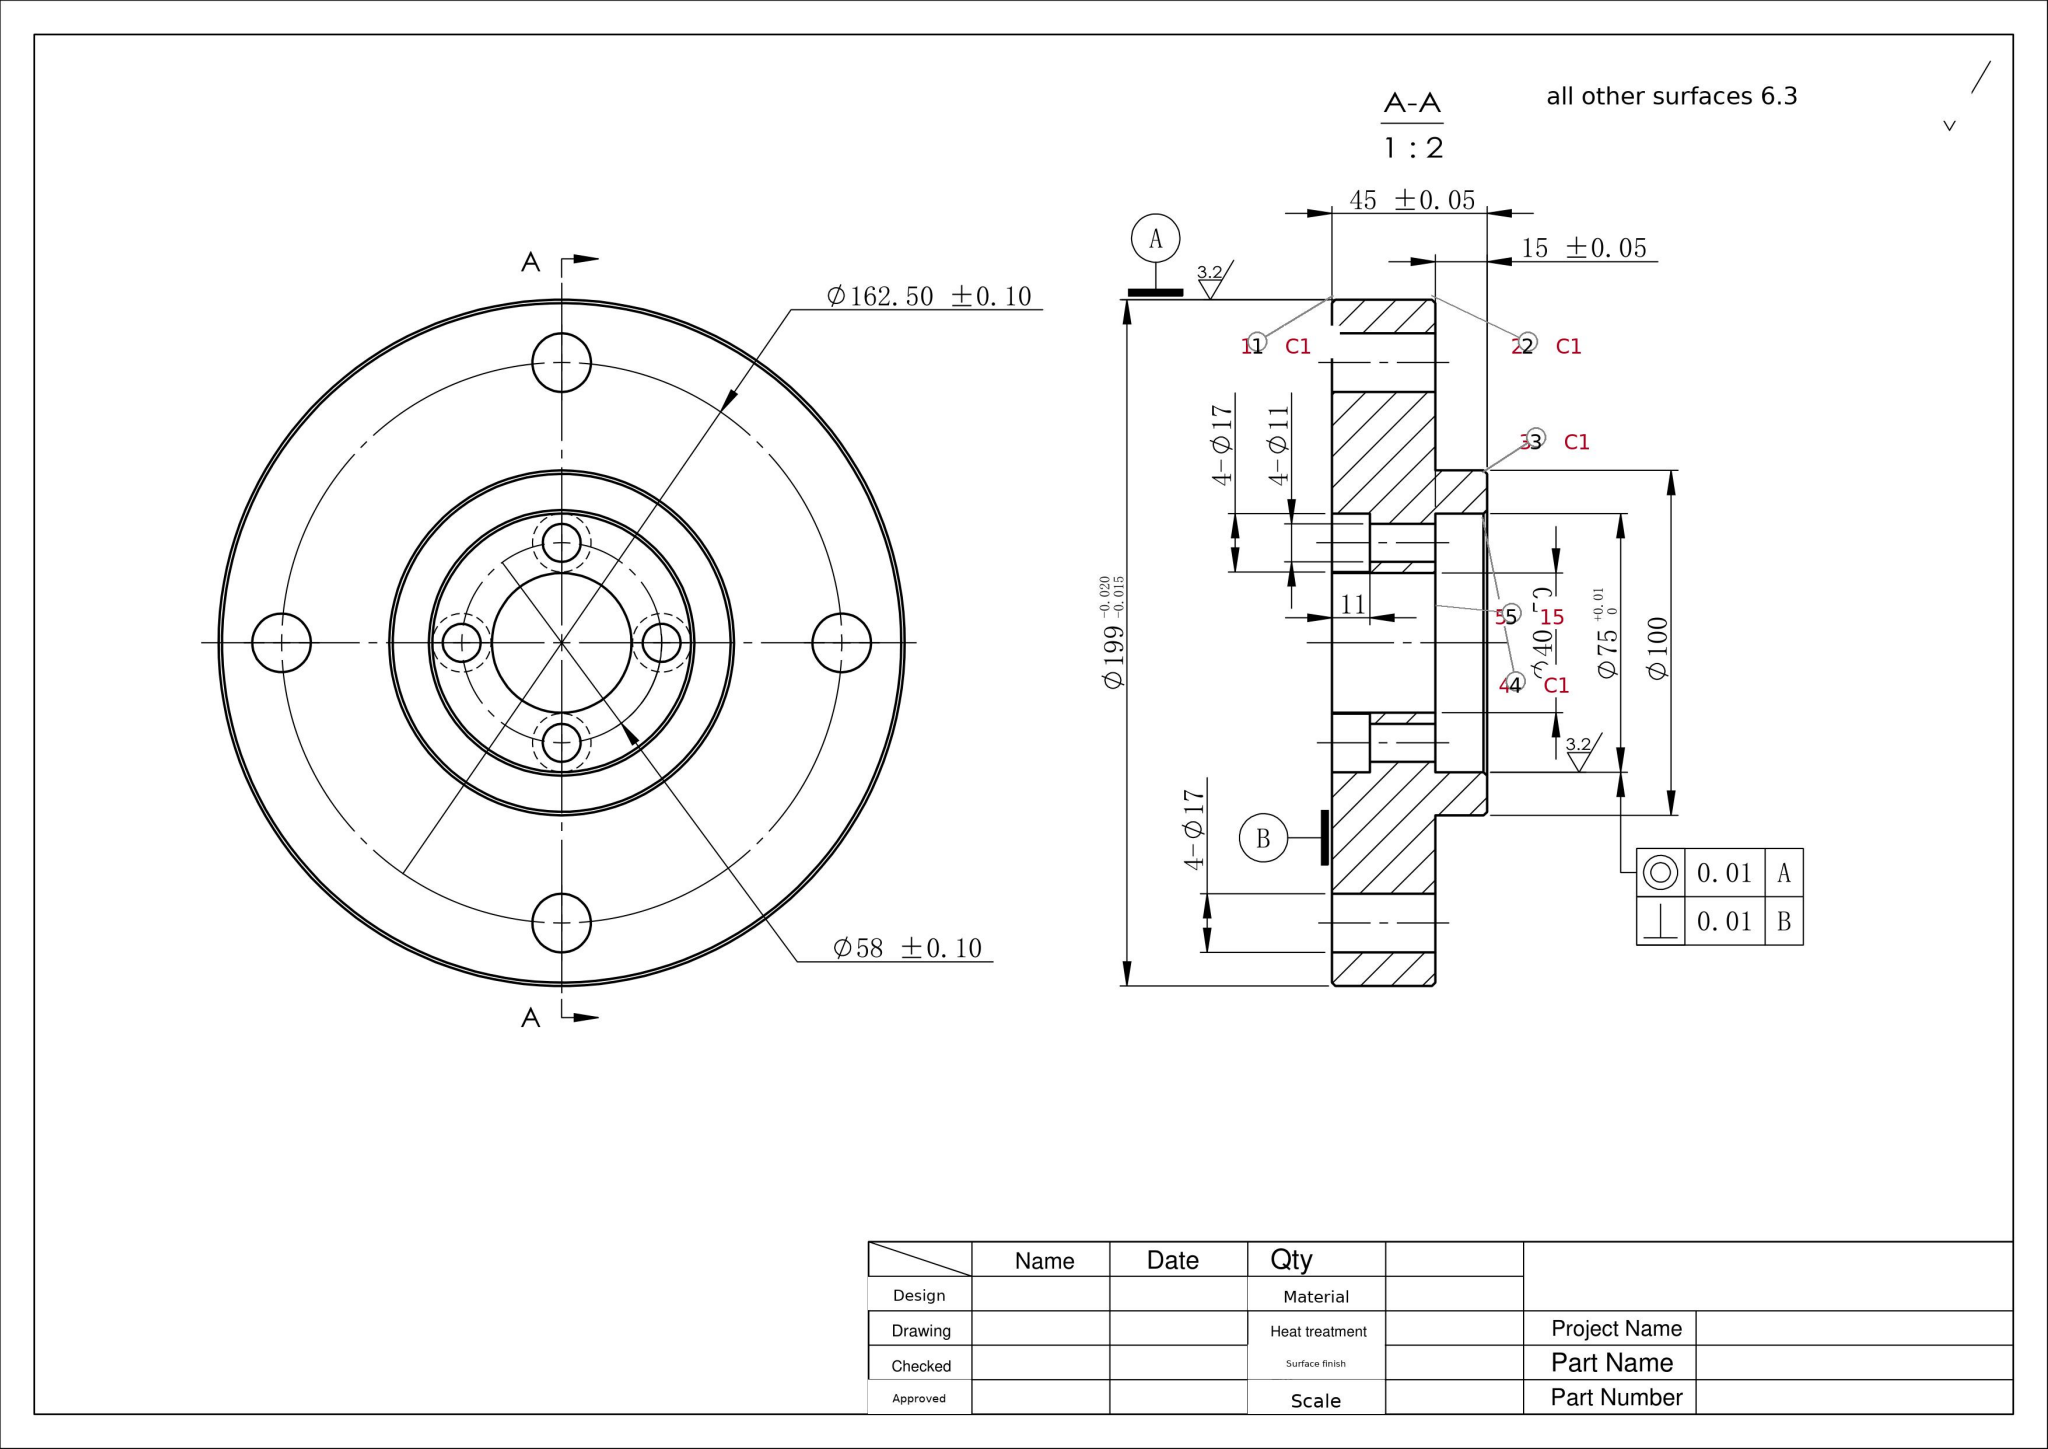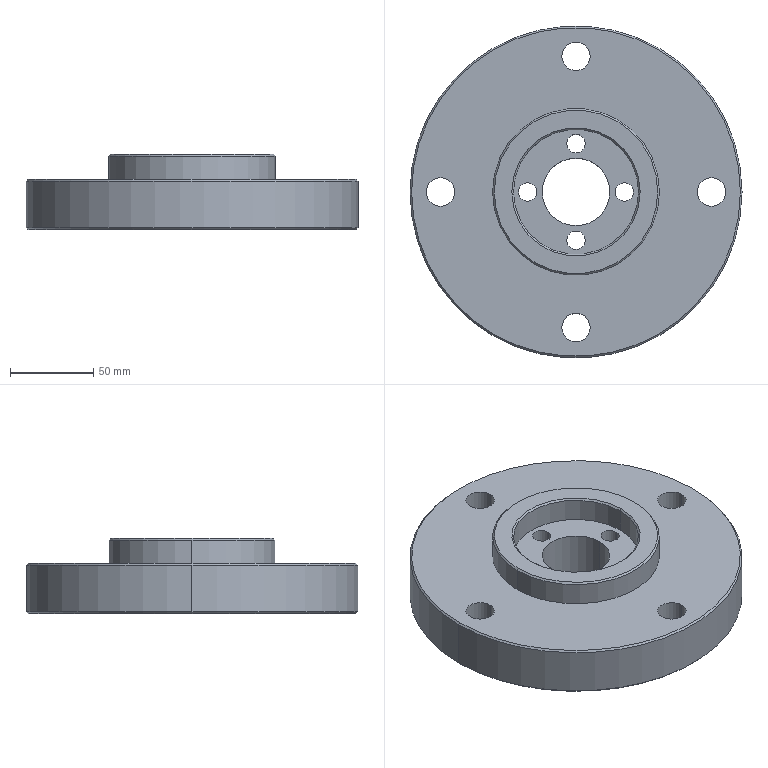Part | SolidWorks | mm | 1 solid | 48 faces | box 199 x 199 x 45 mm | volume 900626 mm3 | cylinder 32 | cone 8 | plane 8 | commonest cylinder face diameters 17 x16 11 x8 40.5 x2 75 x2 100 x2 199 x2
build123d program:
from build123d import *

# Parameters (mm, degrees)
SKETCH1_R          = 99.5
EXTRUDE1_DEPTH     = 30
SKETCH2_R          = 50
SKETCH2_R_2        = 37.5
EXTRUDE2_DEPTH     = 15
SKETCH3_R          = 20.25
CUT_EXTRUDE1_DEPTH = 144.877
SKETCH4_R          = 5.5
CUT_EXTRUDE2_DEPTH = 144.877
CIRPATTERN1_COUNT  = 4
SKETCH5_R          = 8.5
CUT_EXTRUDE3_DEPTH = 144.877
CIRPATTERN2_COUNT  = 4
SKETCH8_R          = 8.5
CUT_EXTRUDE5_DEPTH = 11
CHAMFER1_SIZE      = 1


with BuildPart() as part:
    # Sketch1 → Extrude1 (new body)
    with BuildSketch(Plane.XY):
        Circle(SKETCH1_R)
    extrude(amount=EXTRUDE1_DEPTH)

    # Sketch2 → Extrude2 (add)
    with BuildSketch(Plane.XY.offset(30)):
        Circle(SKETCH2_R)
        Circle(SKETCH2_R_2, mode=Mode.SUBTRACT)
    extrude(amount=EXTRUDE2_DEPTH)

    # Sketch3 → Cut-Extrude1 (cut, through all)
    with BuildSketch(Plane.XY.offset(30)):
        Circle(SKETCH3_R)
    extrude(amount=-CUT_EXTRUDE1_DEPTH, mode=Mode.SUBTRACT)

    # Sketch4 → Cut-Extrude2 (cut, through all)
    with BuildSketch(Plane.XY.offset(30)):
        with Locations((0, 29)):
            Circle(SKETCH4_R)
    cut_extrude2 = extrude(amount=-CUT_EXTRUDE2_DEPTH, mode=Mode.SUBTRACT)

    # CirPattern1: Cut-Extrude2 ×4 about axis
    cirpattern1_axis = Axis((0, 0, 0), (0, 0, 1))
    for i in range(1, CIRPATTERN1_COUNT):
        add(cut_extrude2.rotate(cirpattern1_axis, i * 360 / CIRPATTERN1_COUNT), mode=Mode.SUBTRACT)

    # Sketch5 → Cut-Extrude3 (cut, through all)
    with BuildSketch(Plane.XY.offset(30)):
        with Locations((0, 81.25)):
            Circle(SKETCH5_R)
    cut_extrude3 = extrude(amount=-CUT_EXTRUDE3_DEPTH, mode=Mode.SUBTRACT)

    # CirPattern2: Cut-Extrude3 ×4 about axis
    cirpattern2_axis = Axis((0, 0, 0), (0, 0, 1))
    for i in range(1, CIRPATTERN2_COUNT):
        add(cut_extrude3.rotate(cirpattern2_axis, i * 360 / CIRPATTERN2_COUNT), mode=Mode.SUBTRACT)

    # Sketch8 → Cut-Extrude5 (cut)
    with BuildSketch(Plane(origin=(0, 0, 0), x_dir=(-1, 0, 0), z_dir=(0, 0, -1))):
        with Locations((0, 29)):
            Circle(SKETCH8_R)
        with Locations((-29, 0)):
            Circle(SKETCH8_R)
        with Locations((29, 0)):
            Circle(SKETCH8_R)
        with Locations((0, -29)):
            Circle(SKETCH8_R)
    extrude(amount=-CUT_EXTRUDE5_DEPTH, mode=Mode.SUBTRACT)

    # Chamfer1
    chamfer1_edges = [part.edges().sort_by_distance(p)[0] for p in [
        (-99.5, 0, 0),
        (-99.5, 0, 30),
        (-50, 0, 45),
        (-37.5, 0, 45),
    ]]
    chamfer(chamfer1_edges, length=CHAMFER1_SIZE)


solid = part.part